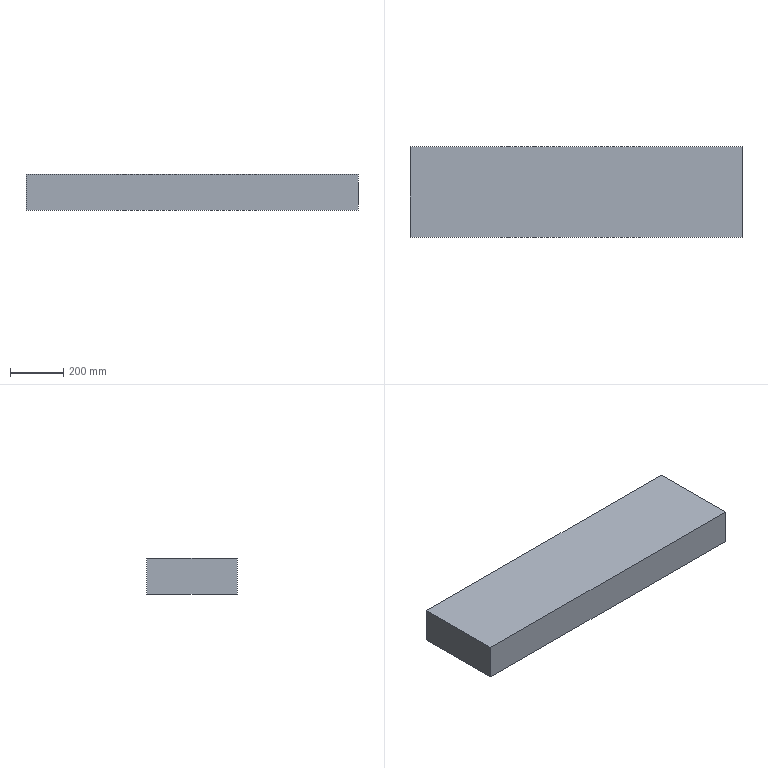Component | NX | CARTON_11 | 1 solid | 13 faces | box 1245 x 340 x 135 mm | volume 6201750 mm3 | plane 13
STEP:
#1=CARTESIAN_POINT('',(0.,0.,0.));
#2=DIRECTION('',(0.,0.,1.));
#3=DIRECTION('',(1.,0.,0.));
#4=AXIS2_PLACEMENT_3D('',#1,#2,#3);
#5=CARTESIAN_POINT('',(622.5,-170.,420.));
#6=VERTEX_POINT('',#5);
#7=CARTESIAN_POINT('',(622.5,170.,420.));
#8=VERTEX_POINT('',#7);
#9=CARTESIAN_POINT('',(622.5,0.,420.));
#10=DIRECTION('',(0.,1.,0.));
#11=VECTOR('',#10,1.);
#12=LINE('',#9,#11);
#13=CARTESIAN_POINT('',(622.5,0.,420.));
#14=DIRECTION('',(1.,0.,0.));
#15=DIRECTION('',(0.,0.,-1.));
#16=AXIS2_PLACEMENT_3D('',#13,#14,#15);
#17=PLANE('',#16);
#18=CARTESIAN_POINT('',(0.,0.));
#19=DIRECTION('',(0.,1.));
#20=VECTOR('',#19,1.);
#21=LINE('',#18,#20);
#22=(GEOMETRIC_REPRESENTATION_CONTEXT(2)PARAMETRIC_REPRESENTATION_CONTEXT()REPRESENTATION_CONTEXT('',''));
#23=DEFINITIONAL_REPRESENTATION('',(#21),#22);
#24=PCURVE('',#17,#23);
#25=CARTESIAN_POINT('',(0.,0.,420.));
#26=DIRECTION('',(0.,0.,-1.));
#27=DIRECTION('',(-1.,0.,0.));
#28=AXIS2_PLACEMENT_3D('',#25,#26,#27);
#29=PLANE('',#28);
#30=CARTESIAN_POINT('',(-622.5,0.));
#31=DIRECTION('',(0.,1.));
#32=VECTOR('',#31,1.);
#33=LINE('',#30,#32);
#34=(GEOMETRIC_REPRESENTATION_CONTEXT(2)PARAMETRIC_REPRESENTATION_CONTEXT()REPRESENTATION_CONTEXT('',''));
#35=DEFINITIONAL_REPRESENTATION('',(#33),#34);
#36=PCURVE('',#29,#35);
#37=SURFACE_CURVE('',#12,(#24,#36),.PCURVE_S1.);
#38=EDGE_CURVE('',#6,#8,#37,.T.);
#39=ORIENTED_EDGE('',*,*,#38,.T.);
#40=CARTESIAN_POINT('',(622.5,170.,555.));
#41=VERTEX_POINT('',#40);
#42=CARTESIAN_POINT('',(622.5,170.,420.));
#43=DIRECTION('',(0.,0.,1.));
#44=VECTOR('',#43,1.);
#45=LINE('',#42,#44);
#46=CARTESIAN_POINT('',(0.,170.));
#47=DIRECTION('',(-1.,0.));
#48=VECTOR('',#47,1.);
#49=LINE('',#46,#48);
#50=(GEOMETRIC_REPRESENTATION_CONTEXT(2)PARAMETRIC_REPRESENTATION_CONTEXT()REPRESENTATION_CONTEXT('',''));
#51=DEFINITIONAL_REPRESENTATION('',(#49),#50);
#52=PCURVE('',#17,#51);
#53=CARTESIAN_POINT('',(0.,170.,420.));
#54=DIRECTION('',(0.,1.,0.));
#55=DIRECTION('',(0.,0.,1.));
#56=AXIS2_PLACEMENT_3D('',#53,#54,#55);
#57=PLANE('',#56);
#58=CARTESIAN_POINT('',(0.,622.5));
#59=DIRECTION('',(1.,0.));
#60=VECTOR('',#59,1.);
#61=LINE('',#58,#60);
#62=(GEOMETRIC_REPRESENTATION_CONTEXT(2)PARAMETRIC_REPRESENTATION_CONTEXT()REPRESENTATION_CONTEXT('',''));
#63=DEFINITIONAL_REPRESENTATION('',(#61),#62);
#64=PCURVE('',#57,#63);
#65=SURFACE_CURVE('',#45,(#52,#64),.PCURVE_S1.);
#66=EDGE_CURVE('',#8,#41,#65,.T.);
#67=ORIENTED_EDGE('',*,*,#66,.T.);
#68=CARTESIAN_POINT('',(622.5,-170.,555.));
#69=VERTEX_POINT('',#68);
#70=CARTESIAN_POINT('',(622.5,0.,555.));
#71=DIRECTION('',(0.,-1.,0.));
#72=VECTOR('',#71,1.);
#73=LINE('',#70,#72);
#74=CARTESIAN_POINT('',(-135.,0.));
#75=DIRECTION('',(0.,-1.));
#76=VECTOR('',#75,1.);
#77=LINE('',#74,#76);
#78=(GEOMETRIC_REPRESENTATION_CONTEXT(2)PARAMETRIC_REPRESENTATION_CONTEXT()REPRESENTATION_CONTEXT('',''));
#79=DEFINITIONAL_REPRESENTATION('',(#77),#78);
#80=PCURVE('',#17,#79);
#81=CARTESIAN_POINT('',(0.,0.,555.));
#82=DIRECTION('',(0.,0.,1.));
#83=DIRECTION('',(1.,0.,0.));
#84=AXIS2_PLACEMENT_3D('',#81,#82,#83);
#85=PLANE('',#84);
#86=CARTESIAN_POINT('',(622.5,0.));
#87=DIRECTION('',(0.,-1.));
#88=VECTOR('',#87,1.);
#89=LINE('',#86,#88);
#90=(GEOMETRIC_REPRESENTATION_CONTEXT(2)PARAMETRIC_REPRESENTATION_CONTEXT()REPRESENTATION_CONTEXT('',''));
#91=DEFINITIONAL_REPRESENTATION('',(#89),#90);
#92=PCURVE('',#85,#91);
#93=SURFACE_CURVE('',#73,(#80,#92),.PCURVE_S1.);
#94=EDGE_CURVE('',#41,#69,#93,.T.);
#95=ORIENTED_EDGE('',*,*,#94,.T.);
#96=CARTESIAN_POINT('',(622.5,-170.,420.));
#97=DIRECTION('',(0.,0.,1.));
#98=VECTOR('',#97,1.);
#99=LINE('',#96,#98);
#100=CARTESIAN_POINT('',(0.,-170.));
#101=DIRECTION('',(-1.,0.));
#102=VECTOR('',#101,1.);
#103=LINE('',#100,#102);
#104=(GEOMETRIC_REPRESENTATION_CONTEXT(2)PARAMETRIC_REPRESENTATION_CONTEXT()REPRESENTATION_CONTEXT('',''));
#105=DEFINITIONAL_REPRESENTATION('',(#103),#104);
#106=PCURVE('',#17,#105);
#107=CARTESIAN_POINT('',(0.,-170.,420.));
#108=DIRECTION('',(0.,-1.,0.));
#109=DIRECTION('',(0.,0.,-1.));
#110=AXIS2_PLACEMENT_3D('',#107,#108,#109);
#111=PLANE('',#110);
#112=CARTESIAN_POINT('',(0.,622.5));
#113=DIRECTION('',(-1.,0.));
#114=VECTOR('',#113,1.);
#115=LINE('',#112,#114);
#116=(GEOMETRIC_REPRESENTATION_CONTEXT(2)PARAMETRIC_REPRESENTATION_CONTEXT()REPRESENTATION_CONTEXT('',''));
#117=DEFINITIONAL_REPRESENTATION('',(#115),#116);
#118=PCURVE('',#111,#117);
#119=SURFACE_CURVE('',#99,(#106,#118),.PCURVE_S1.);
#120=EDGE_CURVE('',#6,#69,#119,.T.);
#121=ORIENTED_EDGE('',*,*,#120,.F.);
#122=EDGE_LOOP('',(#39,#67,#95,#121));
#123=FACE_BOUND('',#122,.T.);
#124=CARTESIAN_POINT('',(622.5,-50.,525.));
#125=VERTEX_POINT('',#124);
#126=CARTESIAN_POINT('',(622.5,50.,525.));
#127=VERTEX_POINT('',#126);
#128=CARTESIAN_POINT('',(622.5,0.,525.));
#129=DIRECTION('',(0.,1.,0.));
#130=VECTOR('',#129,1.);
#131=LINE('',#128,#130);
#132=CARTESIAN_POINT('',(-105.,0.));
#133=DIRECTION('',(0.,1.));
#134=VECTOR('',#133,1.);
#135=LINE('',#132,#134);
#136=(GEOMETRIC_REPRESENTATION_CONTEXT(2)PARAMETRIC_REPRESENTATION_CONTEXT()REPRESENTATION_CONTEXT('',''));
#137=DEFINITIONAL_REPRESENTATION('',(#135),#136);
#138=PCURVE('',#17,#137);
#139=CARTESIAN_POINT('',(622.5,0.,420.));
#140=DIRECTION('',(1.,0.,0.));
#141=DIRECTION('',(0.,0.,-1.));
#142=AXIS2_PLACEMENT_3D('',#139,#140,#141);
#143=PLANE('',#142);
#144=CARTESIAN_POINT('',(-105.,0.));
#145=DIRECTION('',(0.,1.));
#146=VECTOR('',#145,1.);
#147=LINE('',#144,#146);
#148=(GEOMETRIC_REPRESENTATION_CONTEXT(2)PARAMETRIC_REPRESENTATION_CONTEXT()REPRESENTATION_CONTEXT('',''));
#149=DEFINITIONAL_REPRESENTATION('',(#147),#148);
#150=PCURVE('',#143,#149);
#151=SURFACE_CURVE('',#131,(#138,#150),.PCURVE_S1.);
#152=EDGE_CURVE('',#125,#127,#151,.T.);
#153=ORIENTED_EDGE('',*,*,#152,.T.);
#154=CARTESIAN_POINT('',(622.5,50.,445.));
#155=VERTEX_POINT('',#154);
#156=CARTESIAN_POINT('',(622.5,50.,485.));
#157=DIRECTION('',(0.,0.,-1.));
#158=VECTOR('',#157,1.);
#159=LINE('',#156,#158);
#160=CARTESIAN_POINT('',(-65.,50.));
#161=DIRECTION('',(1.,0.));
#162=VECTOR('',#161,1.);
#163=LINE('',#160,#162);
#164=(GEOMETRIC_REPRESENTATION_CONTEXT(2)PARAMETRIC_REPRESENTATION_CONTEXT()REPRESENTATION_CONTEXT('',''));
#165=DEFINITIONAL_REPRESENTATION('',(#163),#164);
#166=PCURVE('',#17,#165);
#167=CARTESIAN_POINT('',(-65.,50.));
#168=DIRECTION('',(1.,0.));
#169=VECTOR('',#168,1.);
#170=LINE('',#167,#169);
#171=(GEOMETRIC_REPRESENTATION_CONTEXT(2)PARAMETRIC_REPRESENTATION_CONTEXT()REPRESENTATION_CONTEXT('',''));
#172=DEFINITIONAL_REPRESENTATION('',(#170),#171);
#173=PCURVE('',#143,#172);
#174=SURFACE_CURVE('',#159,(#166,#173),.PCURVE_S1.);
#175=EDGE_CURVE('',#127,#155,#174,.T.);
#176=ORIENTED_EDGE('',*,*,#175,.T.);
#177=CARTESIAN_POINT('',(622.5,-50.,445.));
#178=VERTEX_POINT('',#177);
#179=CARTESIAN_POINT('',(622.5,0.,445.));
#180=DIRECTION('',(0.,-1.,0.));
#181=VECTOR('',#180,1.);
#182=LINE('',#179,#181);
#183=CARTESIAN_POINT('',(-25.,0.));
#184=DIRECTION('',(0.,-1.));
#185=VECTOR('',#184,1.);
#186=LINE('',#183,#185);
#187=(GEOMETRIC_REPRESENTATION_CONTEXT(2)PARAMETRIC_REPRESENTATION_CONTEXT()REPRESENTATION_CONTEXT('',''));
#188=DEFINITIONAL_REPRESENTATION('',(#186),#187);
#189=PCURVE('',#17,#188);
#190=CARTESIAN_POINT('',(-25.,0.));
#191=DIRECTION('',(0.,-1.));
#192=VECTOR('',#191,1.);
#193=LINE('',#190,#192);
#194=(GEOMETRIC_REPRESENTATION_CONTEXT(2)PARAMETRIC_REPRESENTATION_CONTEXT()REPRESENTATION_CONTEXT('',''));
#195=DEFINITIONAL_REPRESENTATION('',(#193),#194);
#196=PCURVE('',#143,#195);
#197=SURFACE_CURVE('',#182,(#189,#196),.PCURVE_S1.);
#198=EDGE_CURVE('',#155,#178,#197,.T.);
#199=ORIENTED_EDGE('',*,*,#198,.T.);
#200=CARTESIAN_POINT('',(622.5,-50.,485.));
#201=DIRECTION('',(0.,0.,1.));
#202=VECTOR('',#201,1.);
#203=LINE('',#200,#202);
#204=CARTESIAN_POINT('',(-65.,-50.));
#205=DIRECTION('',(-1.,0.));
#206=VECTOR('',#205,1.);
#207=LINE('',#204,#206);
#208=(GEOMETRIC_REPRESENTATION_CONTEXT(2)PARAMETRIC_REPRESENTATION_CONTEXT()REPRESENTATION_CONTEXT('',''));
#209=DEFINITIONAL_REPRESENTATION('',(#207),#208);
#210=PCURVE('',#17,#209);
#211=CARTESIAN_POINT('',(-65.,-50.));
#212=DIRECTION('',(-1.,0.));
#213=VECTOR('',#212,1.);
#214=LINE('',#211,#213);
#215=(GEOMETRIC_REPRESENTATION_CONTEXT(2)PARAMETRIC_REPRESENTATION_CONTEXT()REPRESENTATION_CONTEXT('',''));
#216=DEFINITIONAL_REPRESENTATION('',(#214),#215);
#217=PCURVE('',#143,#216);
#218=SURFACE_CURVE('',#203,(#210,#217),.PCURVE_S1.);
#219=EDGE_CURVE('',#178,#125,#218,.T.);
#220=ORIENTED_EDGE('',*,*,#219,.T.);
#221=EDGE_LOOP('',(#153,#176,#199,#220));
#222=FACE_BOUND('',#221,.T.);
#223=ADVANCED_FACE('',(#123,#222),#17,.T.);
#224=CARTESIAN_POINT('',(-622.5,-170.,555.));
#225=VERTEX_POINT('',#224);
#226=CARTESIAN_POINT('',(0.,-170.,555.));
#227=DIRECTION('',(-1.,0.,0.));
#228=VECTOR('',#227,1.);
#229=LINE('',#226,#228);
#230=CARTESIAN_POINT('',(0.,-170.));
#231=DIRECTION('',(-1.,0.));
#232=VECTOR('',#231,1.);
#233=LINE('',#230,#232);
#234=(GEOMETRIC_REPRESENTATION_CONTEXT(2)PARAMETRIC_REPRESENTATION_CONTEXT()REPRESENTATION_CONTEXT('',''));
#235=DEFINITIONAL_REPRESENTATION('',(#233),#234);
#236=PCURVE('',#85,#235);
#237=CARTESIAN_POINT('',(-135.,0.));
#238=DIRECTION('',(0.,-1.));
#239=VECTOR('',#238,1.);
#240=LINE('',#237,#239);
#241=(GEOMETRIC_REPRESENTATION_CONTEXT(2)PARAMETRIC_REPRESENTATION_CONTEXT()REPRESENTATION_CONTEXT('',''));
#242=DEFINITIONAL_REPRESENTATION('',(#240),#241);
#243=PCURVE('',#111,#242);
#244=SURFACE_CURVE('',#229,(#236,#243),.PCURVE_S1.);
#245=EDGE_CURVE('',#69,#225,#244,.T.);
#246=ORIENTED_EDGE('',*,*,#245,.F.);
#247=ORIENTED_EDGE('',*,*,#94,.F.);
#248=CARTESIAN_POINT('',(-622.5,170.,555.));
#249=VERTEX_POINT('',#248);
#250=CARTESIAN_POINT('',(0.,170.,555.));
#251=DIRECTION('',(1.,0.,0.));
#252=VECTOR('',#251,1.);
#253=LINE('',#250,#252);
#254=CARTESIAN_POINT('',(0.,170.));
#255=DIRECTION('',(1.,0.));
#256=VECTOR('',#255,1.);
#257=LINE('',#254,#256);
#258=(GEOMETRIC_REPRESENTATION_CONTEXT(2)PARAMETRIC_REPRESENTATION_CONTEXT()REPRESENTATION_CONTEXT('',''));
#259=DEFINITIONAL_REPRESENTATION('',(#257),#258);
#260=PCURVE('',#85,#259);
#261=CARTESIAN_POINT('',(135.,0.));
#262=DIRECTION('',(0.,1.));
#263=VECTOR('',#262,1.);
#264=LINE('',#261,#263);
#265=(GEOMETRIC_REPRESENTATION_CONTEXT(2)PARAMETRIC_REPRESENTATION_CONTEXT()REPRESENTATION_CONTEXT('',''));
#266=DEFINITIONAL_REPRESENTATION('',(#264),#265);
#267=PCURVE('',#57,#266);
#268=SURFACE_CURVE('',#253,(#260,#267),.PCURVE_S1.);
#269=EDGE_CURVE('',#249,#41,#268,.T.);
#270=ORIENTED_EDGE('',*,*,#269,.F.);
#271=CARTESIAN_POINT('',(-622.5,0.,555.));
#272=DIRECTION('',(0.,1.,0.));
#273=VECTOR('',#272,1.);
#274=LINE('',#271,#273);
#275=CARTESIAN_POINT('',(-622.5,0.));
#276=DIRECTION('',(0.,1.));
#277=VECTOR('',#276,1.);
#278=LINE('',#275,#277);
#279=(GEOMETRIC_REPRESENTATION_CONTEXT(2)PARAMETRIC_REPRESENTATION_CONTEXT()REPRESENTATION_CONTEXT('',''));
#280=DEFINITIONAL_REPRESENTATION('',(#278),#279);
#281=PCURVE('',#85,#280);
#282=CARTESIAN_POINT('',(-622.5,0.,420.));
#283=DIRECTION('',(-1.,0.,0.));
#284=DIRECTION('',(0.,0.,1.));
#285=AXIS2_PLACEMENT_3D('',#282,#283,#284);
#286=PLANE('',#285);
#287=CARTESIAN_POINT('',(135.,0.));
#288=DIRECTION('',(0.,1.));
#289=VECTOR('',#288,1.);
#290=LINE('',#287,#289);
#291=(GEOMETRIC_REPRESENTATION_CONTEXT(2)PARAMETRIC_REPRESENTATION_CONTEXT()REPRESENTATION_CONTEXT('',''));
#292=DEFINITIONAL_REPRESENTATION('',(#290),#291);
#293=PCURVE('',#286,#292);
#294=SURFACE_CURVE('',#274,(#281,#293),.PCURVE_S1.);
#295=EDGE_CURVE('',#225,#249,#294,.T.);
#296=ORIENTED_EDGE('',*,*,#295,.F.);
#297=EDGE_LOOP('',(#246,#247,#270,#296));
#298=FACE_BOUND('',#297,.T.);
#299=ADVANCED_FACE('',(#298),#85,.T.);
#300=ORIENTED_EDGE('',*,*,#120,.T.);
#301=ORIENTED_EDGE('',*,*,#245,.T.);
#302=CARTESIAN_POINT('',(-622.5,-170.,420.));
#303=VERTEX_POINT('',#302);
#304=CARTESIAN_POINT('',(-622.5,-170.,420.));
#305=DIRECTION('',(0.,0.,1.));
#306=VECTOR('',#305,1.);
#307=LINE('',#304,#306);
#308=CARTESIAN_POINT('',(0.,-622.5));
#309=DIRECTION('',(-1.,0.));
#310=VECTOR('',#309,1.);
#311=LINE('',#308,#310);
#312=(GEOMETRIC_REPRESENTATION_CONTEXT(2)PARAMETRIC_REPRESENTATION_CONTEXT()REPRESENTATION_CONTEXT('',''));
#313=DEFINITIONAL_REPRESENTATION('',(#311),#312);
#314=PCURVE('',#111,#313);
#315=CARTESIAN_POINT('',(0.,-170.));
#316=DIRECTION('',(1.,0.));
#317=VECTOR('',#316,1.);
#318=LINE('',#315,#317);
#319=(GEOMETRIC_REPRESENTATION_CONTEXT(2)PARAMETRIC_REPRESENTATION_CONTEXT()REPRESENTATION_CONTEXT('',''));
#320=DEFINITIONAL_REPRESENTATION('',(#318),#319);
#321=PCURVE('',#286,#320);
#322=SURFACE_CURVE('',#307,(#314,#321),.PCURVE_S1.);
#323=EDGE_CURVE('',#303,#225,#322,.T.);
#324=ORIENTED_EDGE('',*,*,#323,.F.);
#325=CARTESIAN_POINT('',(0.,-170.,420.));
#326=DIRECTION('',(1.,0.,0.));
#327=VECTOR('',#326,1.);
#328=LINE('',#325,#327);
#329=CARTESIAN_POINT('',(0.,0.));
#330=DIRECTION('',(0.,1.));
#331=VECTOR('',#330,1.);
#332=LINE('',#329,#331);
#333=(GEOMETRIC_REPRESENTATION_CONTEXT(2)PARAMETRIC_REPRESENTATION_CONTEXT()REPRESENTATION_CONTEXT('',''));
#334=DEFINITIONAL_REPRESENTATION('',(#332),#333);
#335=PCURVE('',#111,#334);
#336=CARTESIAN_POINT('',(0.,-170.));
#337=DIRECTION('',(-1.,0.));
#338=VECTOR('',#337,1.);
#339=LINE('',#336,#338);
#340=(GEOMETRIC_REPRESENTATION_CONTEXT(2)PARAMETRIC_REPRESENTATION_CONTEXT()REPRESENTATION_CONTEXT('',''));
#341=DEFINITIONAL_REPRESENTATION('',(#339),#340);
#342=PCURVE('',#29,#341);
#343=SURFACE_CURVE('',#328,(#335,#342),.PCURVE_S1.);
#344=EDGE_CURVE('',#303,#6,#343,.T.);
#345=ORIENTED_EDGE('',*,*,#344,.T.);
#346=EDGE_LOOP('',(#300,#301,#324,#345));
#347=FACE_BOUND('',#346,.T.);
#348=ADVANCED_FACE('',(#347),#111,.T.);
#349=ORIENTED_EDGE('',*,*,#323,.T.);
#350=ORIENTED_EDGE('',*,*,#295,.T.);
#351=CARTESIAN_POINT('',(-622.5,170.,420.));
#352=VERTEX_POINT('',#351);
#353=CARTESIAN_POINT('',(-622.5,170.,420.));
#354=DIRECTION('',(0.,0.,1.));
#355=VECTOR('',#354,1.);
#356=LINE('',#353,#355);
#357=CARTESIAN_POINT('',(0.,170.));
#358=DIRECTION('',(1.,0.));
#359=VECTOR('',#358,1.);
#360=LINE('',#357,#359);
#361=(GEOMETRIC_REPRESENTATION_CONTEXT(2)PARAMETRIC_REPRESENTATION_CONTEXT()REPRESENTATION_CONTEXT('',''));
#362=DEFINITIONAL_REPRESENTATION('',(#360),#361);
#363=PCURVE('',#286,#362);
#364=CARTESIAN_POINT('',(0.,-622.5));
#365=DIRECTION('',(1.,0.));
#366=VECTOR('',#365,1.);
#367=LINE('',#364,#366);
#368=(GEOMETRIC_REPRESENTATION_CONTEXT(2)PARAMETRIC_REPRESENTATION_CONTEXT()REPRESENTATION_CONTEXT('',''));
#369=DEFINITIONAL_REPRESENTATION('',(#367),#368);
#370=PCURVE('',#57,#369);
#371=SURFACE_CURVE('',#356,(#363,#370),.PCURVE_S1.);
#372=EDGE_CURVE('',#352,#249,#371,.T.);
#373=ORIENTED_EDGE('',*,*,#372,.F.);
#374=CARTESIAN_POINT('',(-622.5,0.,420.));
#375=DIRECTION('',(0.,-1.,0.));
#376=VECTOR('',#375,1.);
#377=LINE('',#374,#376);
#378=CARTESIAN_POINT('',(0.,0.));
#379=DIRECTION('',(0.,-1.));
#380=VECTOR('',#379,1.);
#381=LINE('',#378,#380);
#382=(GEOMETRIC_REPRESENTATION_CONTEXT(2)PARAMETRIC_REPRESENTATION_CONTEXT()REPRESENTATION_CONTEXT('',''));
#383=DEFINITIONAL_REPRESENTATION('',(#381),#382);
#384=PCURVE('',#286,#383);
#385=CARTESIAN_POINT('',(622.5,0.));
#386=DIRECTION('',(0.,-1.));
#387=VECTOR('',#386,1.);
#388=LINE('',#385,#387);
#389=(GEOMETRIC_REPRESENTATION_CONTEXT(2)PARAMETRIC_REPRESENTATION_CONTEXT()REPRESENTATION_CONTEXT('',''));
#390=DEFINITIONAL_REPRESENTATION('',(#388),#389);
#391=PCURVE('',#29,#390);
#392=SURFACE_CURVE('',#377,(#384,#391),.PCURVE_S1.);
#393=EDGE_CURVE('',#352,#303,#392,.T.);
#394=ORIENTED_EDGE('',*,*,#393,.T.);
#395=EDGE_LOOP('',(#349,#350,#373,#394));
#396=FACE_BOUND('',#395,.T.);
#397=ADVANCED_FACE('',(#396),#286,.T.);
#398=ORIENTED_EDGE('',*,*,#372,.T.);
#399=ORIENTED_EDGE('',*,*,#269,.T.);
#400=ORIENTED_EDGE('',*,*,#66,.F.);
#401=CARTESIAN_POINT('',(0.,170.,420.));
#402=DIRECTION('',(-1.,0.,0.));
#403=VECTOR('',#402,1.);
#404=LINE('',#401,#403);
#405=CARTESIAN_POINT('',(0.,0.));
#406=DIRECTION('',(0.,-1.));
#407=VECTOR('',#406,1.);
#408=LINE('',#405,#407);
#409=(GEOMETRIC_REPRESENTATION_CONTEXT(2)PARAMETRIC_REPRESENTATION_CONTEXT()REPRESENTATION_CONTEXT('',''));
#410=DEFINITIONAL_REPRESENTATION('',(#408),#409);
#411=PCURVE('',#57,#410);
#412=CARTESIAN_POINT('',(0.,170.));
#413=DIRECTION('',(1.,0.));
#414=VECTOR('',#413,1.);
#415=LINE('',#412,#414);
#416=(GEOMETRIC_REPRESENTATION_CONTEXT(2)PARAMETRIC_REPRESENTATION_CONTEXT()REPRESENTATION_CONTEXT('',''));
#417=DEFINITIONAL_REPRESENTATION('',(#415),#416);
#418=PCURVE('',#29,#417);
#419=SURFACE_CURVE('',#404,(#411,#418),.PCURVE_S1.);
#420=EDGE_CURVE('',#8,#352,#419,.T.);
#421=ORIENTED_EDGE('',*,*,#420,.T.);
#422=EDGE_LOOP('',(#398,#399,#400,#421));
#423=FACE_BOUND('',#422,.T.);
#424=ADVANCED_FACE('',(#423),#57,.T.);
#425=ORIENTED_EDGE('',*,*,#38,.F.);
#426=ORIENTED_EDGE('',*,*,#344,.F.);
#427=ORIENTED_EDGE('',*,*,#393,.F.);
#428=ORIENTED_EDGE('',*,*,#420,.F.);
#429=EDGE_LOOP('',(#425,#426,#427,#428));
#430=FACE_BOUND('',#429,.T.);
#431=ADVANCED_FACE('',(#430),#29,.T.);
#432=ORIENTED_EDGE('',*,*,#175,.F.);
#433=ORIENTED_EDGE('',*,*,#152,.F.);
#434=ORIENTED_EDGE('',*,*,#219,.F.);
#435=ORIENTED_EDGE('',*,*,#198,.F.);
#436=EDGE_LOOP('',(#432,#433,#434,#435));
#437=FACE_BOUND('',#436,.T.);
#438=ADVANCED_FACE('',(#437),#143,.T.);
#439=CLOSED_SHELL('',(#223,#299,#348,#397,#424,#431,#438));
#440=CARTESIAN_POINT('',(617.5,-165.,550.));
#441=VERTEX_POINT('',#440);
#442=CARTESIAN_POINT('',(-617.5,-165.,550.));
#443=VERTEX_POINT('',#442);
#444=CARTESIAN_POINT('',(0.,-165.,550.));
#445=DIRECTION('',(-1.,0.,0.));
#446=VECTOR('',#445,1.);
#447=LINE('',#444,#446);
#448=CARTESIAN_POINT('',(0.,0.,550.));
#449=DIRECTION('',(0.,0.,1.));
#450=DIRECTION('',(1.,0.,0.));
#451=AXIS2_PLACEMENT_3D('',#448,#449,#450);
#452=PLANE('',#451);
#453=CARTESIAN_POINT('',(0.,-165.));
#454=DIRECTION('',(-1.,0.));
#455=VECTOR('',#454,1.);
#456=LINE('',#453,#455);
#457=(GEOMETRIC_REPRESENTATION_CONTEXT(2)PARAMETRIC_REPRESENTATION_CONTEXT()REPRESENTATION_CONTEXT('',''));
#458=DEFINITIONAL_REPRESENTATION('',(#456),#457);
#459=PCURVE('',#452,#458);
#460=CARTESIAN_POINT('',(0.,-165.,420.));
#461=DIRECTION('',(0.,-1.,0.));
#462=DIRECTION('',(0.,0.,-1.));
#463=AXIS2_PLACEMENT_3D('',#460,#461,#462);
#464=PLANE('',#463);
#465=CARTESIAN_POINT('',(-130.,0.));
#466=DIRECTION('',(0.,-1.));
#467=VECTOR('',#466,1.);
#468=LINE('',#465,#467);
#469=(GEOMETRIC_REPRESENTATION_CONTEXT(2)PARAMETRIC_REPRESENTATION_CONTEXT()REPRESENTATION_CONTEXT('',''));
#470=DEFINITIONAL_REPRESENTATION('',(#468),#469);
#471=PCURVE('',#464,#470);
#472=SURFACE_CURVE('',#447,(#459,#471),.PCURVE_S1.);
#473=EDGE_CURVE('',#441,#443,#472,.T.);
#474=ORIENTED_EDGE('',*,*,#473,.T.);
#475=CARTESIAN_POINT('',(-617.5,165.,550.));
#476=VERTEX_POINT('',#475);
#477=CARTESIAN_POINT('',(-617.5,0.,550.));
#478=DIRECTION('',(0.,1.,0.));
#479=VECTOR('',#478,1.);
#480=LINE('',#477,#479);
#481=CARTESIAN_POINT('',(-617.5,0.));
#482=DIRECTION('',(0.,1.));
#483=VECTOR('',#482,1.);
#484=LINE('',#481,#483);
#485=(GEOMETRIC_REPRESENTATION_CONTEXT(2)PARAMETRIC_REPRESENTATION_CONTEXT()REPRESENTATION_CONTEXT('',''));
#486=DEFINITIONAL_REPRESENTATION('',(#484),#485);
#487=PCURVE('',#452,#486);
#488=CARTESIAN_POINT('',(-617.5,0.,420.));
#489=DIRECTION('',(-1.,0.,0.));
#490=DIRECTION('',(0.,0.,1.));
#491=AXIS2_PLACEMENT_3D('',#488,#489,#490);
#492=PLANE('',#491);
#493=CARTESIAN_POINT('',(130.,0.));
#494=DIRECTION('',(0.,1.));
#495=VECTOR('',#494,1.);
#496=LINE('',#493,#495);
#497=(GEOMETRIC_REPRESENTATION_CONTEXT(2)PARAMETRIC_REPRESENTATION_CONTEXT()REPRESENTATION_CONTEXT('',''));
#498=DEFINITIONAL_REPRESENTATION('',(#496),#497);
#499=PCURVE('',#492,#498);
#500=SURFACE_CURVE('',#480,(#487,#499),.PCURVE_S1.);
#501=EDGE_CURVE('',#443,#476,#500,.T.);
#502=ORIENTED_EDGE('',*,*,#501,.T.);
#503=CARTESIAN_POINT('',(617.5,165.,550.));
#504=VERTEX_POINT('',#503);
#505=CARTESIAN_POINT('',(0.,165.,550.));
#506=DIRECTION('',(1.,0.,0.));
#507=VECTOR('',#506,1.);
#508=LINE('',#505,#507);
#509=CARTESIAN_POINT('',(0.,165.));
#510=DIRECTION('',(1.,0.));
#511=VECTOR('',#510,1.);
#512=LINE('',#509,#511);
#513=(GEOMETRIC_REPRESENTATION_CONTEXT(2)PARAMETRIC_REPRESENTATION_CONTEXT()REPRESENTATION_CONTEXT('',''));
#514=DEFINITIONAL_REPRESENTATION('',(#512),#513);
#515=PCURVE('',#452,#514);
#516=CARTESIAN_POINT('',(0.,165.,420.));
#517=DIRECTION('',(0.,1.,0.));
#518=DIRECTION('',(0.,0.,1.));
#519=AXIS2_PLACEMENT_3D('',#516,#517,#518);
#520=PLANE('',#519);
#521=CARTESIAN_POINT('',(130.,0.));
#522=DIRECTION('',(0.,1.));
#523=VECTOR('',#522,1.);
#524=LINE('',#521,#523);
#525=(GEOMETRIC_REPRESENTATION_CONTEXT(2)PARAMETRIC_REPRESENTATION_CONTEXT()REPRESENTATION_CONTEXT('',''));
#526=DEFINITIONAL_REPRESENTATION('',(#524),#525);
#527=PCURVE('',#520,#526);
#528=SURFACE_CURVE('',#508,(#515,#527),.PCURVE_S1.);
#529=EDGE_CURVE('',#476,#504,#528,.T.);
#530=ORIENTED_EDGE('',*,*,#529,.T.);
#531=CARTESIAN_POINT('',(617.5,0.,550.));
#532=DIRECTION('',(0.,-1.,0.));
#533=VECTOR('',#532,1.);
#534=LINE('',#531,#533);
#535=CARTESIAN_POINT('',(617.5,0.));
#536=DIRECTION('',(0.,-1.));
#537=VECTOR('',#536,1.);
#538=LINE('',#535,#537);
#539=(GEOMETRIC_REPRESENTATION_CONTEXT(2)PARAMETRIC_REPRESENTATION_CONTEXT()REPRESENTATION_CONTEXT('',''));
#540=DEFINITIONAL_REPRESENTATION('',(#538),#539);
#541=PCURVE('',#452,#540);
#542=CARTESIAN_POINT('',(617.5,0.,420.));
#543=DIRECTION('',(1.,0.,0.));
#544=DIRECTION('',(0.,0.,-1.));
#545=AXIS2_PLACEMENT_3D('',#542,#543,#544);
#546=PLANE('',#545);
#547=CARTESIAN_POINT('',(-130.,0.));
#548=DIRECTION('',(0.,-1.));
#549=VECTOR('',#548,1.);
#550=LINE('',#547,#549);
#551=(GEOMETRIC_REPRESENTATION_CONTEXT(2)PARAMETRIC_REPRESENTATION_CONTEXT()REPRESENTATION_CONTEXT('',''));
#552=DEFINITIONAL_REPRESENTATION('',(#550),#551);
#553=PCURVE('',#546,#552);
#554=SURFACE_CURVE('',#534,(#541,#553),.PCURVE_S1.);
#555=EDGE_CURVE('',#504,#441,#554,.T.);
#556=ORIENTED_EDGE('',*,*,#555,.T.);
#557=EDGE_LOOP('',(#474,#502,#530,#556));
#558=FACE_BOUND('',#557,.F.);
#559=ADVANCED_FACE('',(#558),#452,.T.);
#560=CARTESIAN_POINT('',(617.5,-165.,425.));
#561=VERTEX_POINT('',#560);
#562=CARTESIAN_POINT('',(617.5,-165.,420.));
#563=DIRECTION('',(0.,0.,1.));
#564=VECTOR('',#563,1.);
#565=LINE('',#562,#564);
#566=CARTESIAN_POINT('',(0.,617.5));
#567=DIRECTION('',(-1.,0.));
#568=VECTOR('',#567,1.);
#569=LINE('',#566,#568);
#570=(GEOMETRIC_REPRESENTATION_CONTEXT(2)PARAMETRIC_REPRESENTATION_CONTEXT()REPRESENTATION_CONTEXT('',''));
#571=DEFINITIONAL_REPRESENTATION('',(#569),#570);
#572=PCURVE('',#464,#571);
#573=CARTESIAN_POINT('',(0.,-165.));
#574=DIRECTION('',(-1.,0.));
#575=VECTOR('',#574,1.);
#576=LINE('',#573,#575);
#577=(GEOMETRIC_REPRESENTATION_CONTEXT(2)PARAMETRIC_REPRESENTATION_CONTEXT()REPRESENTATION_CONTEXT('',''));
#578=DEFINITIONAL_REPRESENTATION('',(#576),#577);
#579=PCURVE('',#546,#578);
#580=SURFACE_CURVE('',#565,(#572,#579),.PCURVE_S1.);
#581=EDGE_CURVE('',#561,#441,#580,.T.);
#582=ORIENTED_EDGE('',*,*,#581,.F.);
#583=CARTESIAN_POINT('',(-617.5,-165.,425.));
#584=VERTEX_POINT('',#583);
#585=CARTESIAN_POINT('',(0.,-165.,425.));
#586=DIRECTION('',(1.,0.,0.));
#587=VECTOR('',#586,1.);
#588=LINE('',#585,#587);
#589=CARTESIAN_POINT('',(-5.,0.));
#590=DIRECTION('',(0.,1.));
#591=VECTOR('',#590,1.);
#592=LINE('',#589,#591);
#593=(GEOMETRIC_REPRESENTATION_CONTEXT(2)PARAMETRIC_REPRESENTATION_CONTEXT()REPRESENTATION_CONTEXT('',''));
#594=DEFINITIONAL_REPRESENTATION('',(#592),#593);
#595=PCURVE('',#464,#594);
#596=CARTESIAN_POINT('',(0.,0.,425.));
#597=DIRECTION('',(0.,0.,-1.));
#598=DIRECTION('',(-1.,0.,0.));
#599=AXIS2_PLACEMENT_3D('',#596,#597,#598);
#600=PLANE('',#599);
#601=CARTESIAN_POINT('',(0.,-165.));
#602=DIRECTION('',(-1.,0.));
#603=VECTOR('',#602,1.);
#604=LINE('',#601,#603);
#605=(GEOMETRIC_REPRESENTATION_CONTEXT(2)PARAMETRIC_REPRESENTATION_CONTEXT()REPRESENTATION_CONTEXT('',''));
#606=DEFINITIONAL_REPRESENTATION('',(#604),#605);
#607=PCURVE('',#600,#606);
#608=SURFACE_CURVE('',#588,(#595,#607),.PCURVE_S1.);
#609=EDGE_CURVE('',#584,#561,#608,.T.);
#610=ORIENTED_EDGE('',*,*,#609,.F.);
#611=CARTESIAN_POINT('',(-617.5,-165.,420.));
#612=DIRECTION('',(0.,0.,1.));
#613=VECTOR('',#612,1.);
#614=LINE('',#611,#613);
#615=CARTESIAN_POINT('',(0.,-617.5));
#616=DIRECTION('',(-1.,0.));
#617=VECTOR('',#616,1.);
#618=LINE('',#615,#617);
#619=(GEOMETRIC_REPRESENTATION_CONTEXT(2)PARAMETRIC_REPRESENTATION_CONTEXT()REPRESENTATION_CONTEXT('',''));
#620=DEFINITIONAL_REPRESENTATION('',(#618),#619);
#621=PCURVE('',#464,#620);
#622=CARTESIAN_POINT('',(0.,-165.));
#623=DIRECTION('',(1.,0.));
#624=VECTOR('',#623,1.);
#625=LINE('',#622,#624);
#626=(GEOMETRIC_REPRESENTATION_CONTEXT(2)PARAMETRIC_REPRESENTATION_CONTEXT()REPRESENTATION_CONTEXT('',''));
#627=DEFINITIONAL_REPRESENTATION('',(#625),#626);
#628=PCURVE('',#492,#627);
#629=SURFACE_CURVE('',#614,(#621,#628),.PCURVE_S1.);
#630=EDGE_CURVE('',#584,#443,#629,.T.);
#631=ORIENTED_EDGE('',*,*,#630,.T.);
#632=ORIENTED_EDGE('',*,*,#473,.F.);
#633=EDGE_LOOP('',(#582,#610,#631,#632));
#634=FACE_BOUND('',#633,.F.);
#635=ADVANCED_FACE('',(#634),#464,.T.);
#636=ORIENTED_EDGE('',*,*,#630,.F.);
#637=CARTESIAN_POINT('',(-617.5,165.,425.));
#638=VERTEX_POINT('',#637);
#639=CARTESIAN_POINT('',(-617.5,0.,425.));
#640=DIRECTION('',(0.,-1.,0.));
#641=VECTOR('',#640,1.);
#642=LINE('',#639,#641);
#643=CARTESIAN_POINT('',(5.,0.));
#644=DIRECTION('',(0.,-1.));
#645=VECTOR('',#644,1.);
#646=LINE('',#643,#645);
#647=(GEOMETRIC_REPRESENTATION_CONTEXT(2)PARAMETRIC_REPRESENTATION_CONTEXT()REPRESENTATION_CONTEXT('',''));
#648=DEFINITIONAL_REPRESENTATION('',(#646),#647);
#649=PCURVE('',#492,#648);
#650=CARTESIAN_POINT('',(617.5,0.));
#651=DIRECTION('',(0.,-1.));
#652=VECTOR('',#651,1.);
#653=LINE('',#650,#652);
#654=(GEOMETRIC_REPRESENTATION_CONTEXT(2)PARAMETRIC_REPRESENTATION_CONTEXT()REPRESENTATION_CONTEXT('',''));
#655=DEFINITIONAL_REPRESENTATION('',(#653),#654);
#656=PCURVE('',#600,#655);
#657=SURFACE_CURVE('',#642,(#649,#656),.PCURVE_S1.);
#658=EDGE_CURVE('',#638,#584,#657,.T.);
#659=ORIENTED_EDGE('',*,*,#658,.F.);
#660=CARTESIAN_POINT('',(-617.5,165.,420.));
#661=DIRECTION('',(0.,0.,1.));
#662=VECTOR('',#661,1.);
#663=LINE('',#660,#662);
#664=CARTESIAN_POINT('',(0.,165.));
#665=DIRECTION('',(1.,0.));
#666=VECTOR('',#665,1.);
#667=LINE('',#664,#666);
#668=(GEOMETRIC_REPRESENTATION_CONTEXT(2)PARAMETRIC_REPRESENTATION_CONTEXT()REPRESENTATION_CONTEXT('',''));
#669=DEFINITIONAL_REPRESENTATION('',(#667),#668);
#670=PCURVE('',#492,#669);
#671=CARTESIAN_POINT('',(0.,-617.5));
#672=DIRECTION('',(1.,0.));
#673=VECTOR('',#672,1.);
#674=LINE('',#671,#673);
#675=(GEOMETRIC_REPRESENTATION_CONTEXT(2)PARAMETRIC_REPRESENTATION_CONTEXT()REPRESENTATION_CONTEXT('',''));
#676=DEFINITIONAL_REPRESENTATION('',(#674),#675);
#677=PCURVE('',#520,#676);
#678=SURFACE_CURVE('',#663,(#670,#677),.PCURVE_S1.);
#679=EDGE_CURVE('',#638,#476,#678,.T.);
#680=ORIENTED_EDGE('',*,*,#679,.T.);
#681=ORIENTED_EDGE('',*,*,#501,.F.);
#682=EDGE_LOOP('',(#636,#659,#680,#681));
#683=FACE_BOUND('',#682,.F.);
#684=ADVANCED_FACE('',(#683),#492,.T.);
#685=ORIENTED_EDGE('',*,*,#679,.F.);
#686=CARTESIAN_POINT('',(617.5,165.,425.));
#687=VERTEX_POINT('',#686);
#688=CARTESIAN_POINT('',(0.,165.,425.));
#689=DIRECTION('',(-1.,0.,0.));
#690=VECTOR('',#689,1.);
#691=LINE('',#688,#690);
#692=CARTESIAN_POINT('',(5.,0.));
#693=DIRECTION('',(0.,-1.));
#694=VECTOR('',#693,1.);
#695=LINE('',#692,#694);
#696=(GEOMETRIC_REPRESENTATION_CONTEXT(2)PARAMETRIC_REPRESENTATION_CONTEXT()REPRESENTATION_CONTEXT('',''));
#697=DEFINITIONAL_REPRESENTATION('',(#695),#696);
#698=PCURVE('',#520,#697);
#699=CARTESIAN_POINT('',(0.,165.));
#700=DIRECTION('',(1.,0.));
#701=VECTOR('',#700,1.);
#702=LINE('',#699,#701);
#703=(GEOMETRIC_REPRESENTATION_CONTEXT(2)PARAMETRIC_REPRESENTATION_CONTEXT()REPRESENTATION_CONTEXT('',''));
#704=DEFINITIONAL_REPRESENTATION('',(#702),#703);
#705=PCURVE('',#600,#704);
#706=SURFACE_CURVE('',#691,(#698,#705),.PCURVE_S1.);
#707=EDGE_CURVE('',#687,#638,#706,.T.);
#708=ORIENTED_EDGE('',*,*,#707,.F.);
#709=CARTESIAN_POINT('',(617.5,165.,420.));
#710=DIRECTION('',(0.,0.,1.));
#711=VECTOR('',#710,1.);
#712=LINE('',#709,#711);
#713=CARTESIAN_POINT('',(0.,617.5));
#714=DIRECTION('',(1.,0.));
#715=VECTOR('',#714,1.);
#716=LINE('',#713,#715);
#717=(GEOMETRIC_REPRESENTATION_CONTEXT(2)PARAMETRIC_REPRESENTATION_CONTEXT()REPRESENTATION_CONTEXT('',''));
#718=DEFINITIONAL_REPRESENTATION('',(#716),#717);
#719=PCURVE('',#520,#718);
#720=CARTESIAN_POINT('',(0.,165.));
#721=DIRECTION('',(-1.,0.));
#722=VECTOR('',#721,1.);
#723=LINE('',#720,#722);
#724=(GEOMETRIC_REPRESENTATION_CONTEXT(2)PARAMETRIC_REPRESENTATION_CONTEXT()REPRESENTATION_CONTEXT('',''));
#725=DEFINITIONAL_REPRESENTATION('',(#723),#724);
#726=PCURVE('',#546,#725);
#727=SURFACE_CURVE('',#712,(#719,#726),.PCURVE_S1.);
#728=EDGE_CURVE('',#687,#504,#727,.T.);
#729=ORIENTED_EDGE('',*,*,#728,.T.);
#730=ORIENTED_EDGE('',*,*,#529,.F.);
#731=EDGE_LOOP('',(#685,#708,#729,#730));
#732=FACE_BOUND('',#731,.F.);
#733=ADVANCED_FACE('',(#732),#520,.T.);
#734=CARTESIAN_POINT('',(617.5,0.,425.));
#735=DIRECTION('',(0.,1.,0.));
#736=VECTOR('',#735,1.);
#737=LINE('',#734,#736);
#738=CARTESIAN_POINT('',(-617.5,0.));
#739=DIRECTION('',(0.,1.));
#740=VECTOR('',#739,1.);
#741=LINE('',#738,#740);
#742=(GEOMETRIC_REPRESENTATION_CONTEXT(2)PARAMETRIC_REPRESENTATION_CONTEXT()REPRESENTATION_CONTEXT('',''));
#743=DEFINITIONAL_REPRESENTATION('',(#741),#742);
#744=PCURVE('',#600,#743);
#745=CARTESIAN_POINT('',(-5.,0.));
#746=DIRECTION('',(0.,1.));
#747=VECTOR('',#746,1.);
#748=LINE('',#745,#747);
#749=(GEOMETRIC_REPRESENTATION_CONTEXT(2)PARAMETRIC_REPRESENTATION_CONTEXT()REPRESENTATION_CONTEXT('',''));
#750=DEFINITIONAL_REPRESENTATION('',(#748),#749);
#751=PCURVE('',#546,#750);
#752=SURFACE_CURVE('',#737,(#744,#751),.PCURVE_S1.);
#753=EDGE_CURVE('',#561,#687,#752,.T.);
#754=ORIENTED_EDGE('',*,*,#753,.T.);
#755=ORIENTED_EDGE('',*,*,#707,.T.);
#756=ORIENTED_EDGE('',*,*,#658,.T.);
#757=ORIENTED_EDGE('',*,*,#609,.T.);
#758=EDGE_LOOP('',(#754,#755,#756,#757));
#759=FACE_BOUND('',#758,.F.);
#760=ADVANCED_FACE('',(#759),#600,.T.);
#761=ORIENTED_EDGE('',*,*,#753,.F.);
#762=ORIENTED_EDGE('',*,*,#581,.T.);
#763=ORIENTED_EDGE('',*,*,#555,.F.);
#764=ORIENTED_EDGE('',*,*,#728,.F.);
#765=EDGE_LOOP('',(#761,#762,#763,#764));
#766=FACE_BOUND('',#765,.F.);
#767=ADVANCED_FACE('',(#766),#546,.T.);
#768=CLOSED_SHELL('',(#559,#635,#684,#733,#760,#767));
#769=ORIENTED_CLOSED_SHELL('',*,#768,.F.);
#770=BREP_WITH_VOIDS('',#439,(#769));
#771=(LENGTH_UNIT()NAMED_UNIT(*)SI_UNIT(.MILLI.,.METRE.));
#772=UNCERTAINTY_MEASURE_WITH_UNIT(LENGTH_MEASURE(0.0000001),#771,'','');
#773=(NAMED_UNIT(*)PLANE_ANGLE_UNIT()SI_UNIT($,.RADIAN.));
#774=(NAMED_UNIT(*)SI_UNIT($,.STERADIAN.)SOLID_ANGLE_UNIT());
#775=(GEOMETRIC_REPRESENTATION_CONTEXT(3)GLOBAL_UNCERTAINTY_ASSIGNED_CONTEXT((#772))GLOBAL_UNIT_ASSIGNED_CONTEXT((#771,#773,#774))REPRESENTATION_CONTEXT('',''));
#776=ADVANCED_BREP_SHAPE_REPRESENTATION('',(#4,#770),#775);